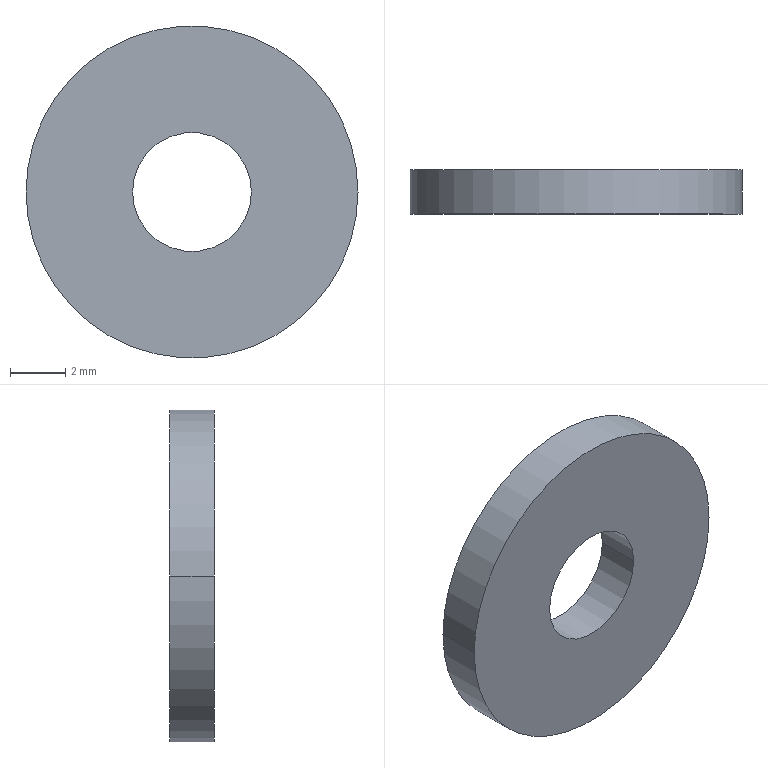Component | SolidWorks | TBN12-4-3 | 1 solid | 6 faces | box 12 x 1.6 x 12 mm | volume 158 mm3 | cylinder 4 | plane 2 | commonest cylinder face diameters 4.3 x2 12 x2
build123d program:
from build123d import *

# Parameters (mm, degrees)
SKETCH1_R           = 6
SKETCH1_R_2         = 2.15
BOSS_EXTRUDE1_DEPTH = 1.6


with BuildPart() as part:
    # Sketch1 → Boss-Extrude1 (new body)
    with BuildSketch(Plane.XY):
        Circle(SKETCH1_R)
        Circle(SKETCH1_R_2, mode=Mode.SUBTRACT)
    extrude(amount=BOSS_EXTRUDE1_DEPTH)


solid = part.part

# Placed as in the assembly
solid = solid.moved(Location((-57.536, 77.85, 217.788), (90, 0, 0)))
STEP:
#1=COLOUR_RGB('',0.7922,0.8196,0.9333);
#2=FILL_AREA_STYLE_COLOUR('',#1);
#3=FILL_AREA_STYLE('',(#2));
#4=SURFACE_STYLE_FILL_AREA(#3);
#5=SURFACE_SIDE_STYLE('',(#4));
#6=SURFACE_STYLE_USAGE(.BOTH.,#5);
#7=PRESENTATION_STYLE_ASSIGNMENT((#6));
#8=CARTESIAN_POINT('',(-2.35,3.002,8.574));
#9=VERTEX_POINT('',#8);
#10=CARTESIAN_POINT('',(-2.181,3.002,8.574));
#11=VERTEX_POINT('',#10);
#12=CARTESIAN_POINT('',(-2.265,3.002,8.574));
#13=DIRECTION('',(0.,-1.,-0.));
#14=DIRECTION('',(1.,0.,0.));
#15=AXIS2_PLACEMENT_3D('',#12,#13,#14);
#16=CIRCLE('',#15,0.08465);
#17=EDGE_CURVE('',#9,#11,#16,.T.);
#18=ORIENTED_EDGE('',*,*,#17,.T.);
#19=CARTESIAN_POINT('',(-2.181,3.065,8.574));
#20=VERTEX_POINT('',#19);
#21=CARTESIAN_POINT('',(-2.181,3.002,8.574));
#22=DIRECTION('',(-0.,1.,0.));
#23=VECTOR('',#22,39.37);
#24=LINE('',#21,#23);
#25=EDGE_CURVE('',#11,#20,#24,.T.);
#26=ORIENTED_EDGE('',*,*,#25,.T.);
#27=CARTESIAN_POINT('',(-2.35,3.065,8.574));
#28=VERTEX_POINT('',#27);
#29=CARTESIAN_POINT('',(-2.265,3.065,8.574));
#30=DIRECTION('',(0.,-1.,-0.));
#31=DIRECTION('',(1.,0.,0.));
#32=AXIS2_PLACEMENT_3D('',#29,#30,#31);
#33=CIRCLE('',#32,0.08465);
#34=EDGE_CURVE('',#28,#20,#33,.T.);
#35=ORIENTED_EDGE('',*,*,#34,.F.);
#36=CARTESIAN_POINT('',(-2.35,3.002,8.574));
#37=DIRECTION('',(-0.,1.,0.));
#38=VECTOR('',#37,39.37);
#39=LINE('',#36,#38);
#40=EDGE_CURVE('',#9,#28,#39,.T.);
#41=ORIENTED_EDGE('',*,*,#40,.F.);
#42=EDGE_LOOP('',(#18,#26,#35,#41));
#43=FACE_OUTER_BOUND('',#42,.T.);
#44=CARTESIAN_POINT('',(-2.265,3.002,8.574));
#45=DIRECTION('',(-0.,1.,0.));
#46=DIRECTION('',(-1.,0.,0.));
#47=AXIS2_PLACEMENT_3D('',#44,#45,#46);
#48=CYLINDRICAL_SURFACE('',#47,0.08465);
#49=ADVANCED_FACE('',(#43),#48,.F.);
#50=CARTESIAN_POINT('',(-2.029,3.002,8.574));
#51=VERTEX_POINT('',#50);
#52=CARTESIAN_POINT('',(-2.501,3.002,8.574));
#53=VERTEX_POINT('',#52);
#54=CARTESIAN_POINT('',(-2.265,3.002,8.574));
#55=DIRECTION('',(0.,-1.,-0.));
#56=DIRECTION('',(1.,0.,0.));
#57=AXIS2_PLACEMENT_3D('',#54,#55,#56);
#58=CIRCLE('',#57,0.2362);
#59=EDGE_CURVE('',#51,#53,#58,.T.);
#60=ORIENTED_EDGE('',*,*,#59,.F.);
#61=CARTESIAN_POINT('',(-2.029,3.065,8.574));
#62=VERTEX_POINT('',#61);
#63=CARTESIAN_POINT('',(-2.029,3.002,8.574));
#64=DIRECTION('',(-0.,1.,0.));
#65=VECTOR('',#64,39.37);
#66=LINE('',#63,#65);
#67=EDGE_CURVE('',#51,#62,#66,.T.);
#68=ORIENTED_EDGE('',*,*,#67,.T.);
#69=CARTESIAN_POINT('',(-2.501,3.065,8.574));
#70=VERTEX_POINT('',#69);
#71=CARTESIAN_POINT('',(-2.265,3.065,8.574));
#72=DIRECTION('',(0.,-1.,-0.));
#73=DIRECTION('',(1.,0.,0.));
#74=AXIS2_PLACEMENT_3D('',#71,#72,#73);
#75=CIRCLE('',#74,0.2362);
#76=EDGE_CURVE('',#62,#70,#75,.T.);
#77=ORIENTED_EDGE('',*,*,#76,.T.);
#78=CARTESIAN_POINT('',(-2.501,3.002,8.574));
#79=DIRECTION('',(-0.,1.,0.));
#80=VECTOR('',#79,39.37);
#81=LINE('',#78,#80);
#82=EDGE_CURVE('',#53,#70,#81,.T.);
#83=ORIENTED_EDGE('',*,*,#82,.F.);
#84=EDGE_LOOP('',(#60,#68,#77,#83));
#85=FACE_OUTER_BOUND('',#84,.T.);
#86=CARTESIAN_POINT('',(-2.265,3.002,8.574));
#87=DIRECTION('',(-0.,1.,0.));
#88=DIRECTION('',(-1.,0.,0.));
#89=AXIS2_PLACEMENT_3D('',#86,#87,#88);
#90=CYLINDRICAL_SURFACE('',#89,0.2362);
#91=ADVANCED_FACE('',(#85),#90,.T.);
#92=CARTESIAN_POINT('',(-2.265,3.002,8.574));
#93=DIRECTION('',(0.,-1.,-0.));
#94=DIRECTION('',(1.,0.,0.));
#95=AXIS2_PLACEMENT_3D('',#92,#93,#94);
#96=CIRCLE('',#95,0.2362);
#97=EDGE_CURVE('',#53,#51,#96,.T.);
#98=ORIENTED_EDGE('',*,*,#97,.T.);
#99=ORIENTED_EDGE('',*,*,#59,.T.);
#100=EDGE_LOOP('',(#98,#99));
#101=FACE_OUTER_BOUND('',#100,.T.);
#102=ORIENTED_EDGE('',*,*,#17,.F.);
#103=CARTESIAN_POINT('',(-2.265,3.002,8.574));
#104=DIRECTION('',(0.,-1.,-0.));
#105=DIRECTION('',(1.,0.,0.));
#106=AXIS2_PLACEMENT_3D('',#103,#104,#105);
#107=CIRCLE('',#106,0.08465);
#108=EDGE_CURVE('',#11,#9,#107,.T.);
#109=ORIENTED_EDGE('',*,*,#108,.F.);
#110=EDGE_LOOP('',(#102,#109));
#111=FACE_BOUND('',#110,.T.);
#112=CARTESIAN_POINT('',(-2.265,3.002,8.574));
#113=DIRECTION('',(0.,-1.,-0.));
#114=DIRECTION('',(1.,0.,-0.));
#115=AXIS2_PLACEMENT_3D('',#112,#113,#114);
#116=PLANE('',#115);
#117=ADVANCED_FACE('',(#101,#111),#116,.T.);
#118=CARTESIAN_POINT('',(-2.265,3.065,8.574));
#119=DIRECTION('',(0.,-1.,-0.));
#120=DIRECTION('',(1.,0.,0.));
#121=AXIS2_PLACEMENT_3D('',#118,#119,#120);
#122=CIRCLE('',#121,0.2362);
#123=EDGE_CURVE('',#70,#62,#122,.T.);
#124=ORIENTED_EDGE('',*,*,#123,.F.);
#125=ORIENTED_EDGE('',*,*,#76,.F.);
#126=EDGE_LOOP('',(#124,#125));
#127=FACE_OUTER_BOUND('',#126,.T.);
#128=ORIENTED_EDGE('',*,*,#34,.T.);
#129=CARTESIAN_POINT('',(-2.265,3.065,8.574));
#130=DIRECTION('',(0.,-1.,-0.));
#131=DIRECTION('',(1.,0.,0.));
#132=AXIS2_PLACEMENT_3D('',#129,#130,#131);
#133=CIRCLE('',#132,0.08465);
#134=EDGE_CURVE('',#20,#28,#133,.T.);
#135=ORIENTED_EDGE('',*,*,#134,.T.);
#136=EDGE_LOOP('',(#128,#135));
#137=FACE_BOUND('',#136,.T.);
#138=CARTESIAN_POINT('',(-2.265,3.065,8.574));
#139=DIRECTION('',(0.,-1.,-0.));
#140=DIRECTION('',(1.,0.,-0.));
#141=AXIS2_PLACEMENT_3D('',#138,#139,#140);
#142=PLANE('',#141);
#143=ADVANCED_FACE('',(#127,#137),#142,.F.);
#144=ORIENTED_EDGE('',*,*,#67,.F.);
#145=ORIENTED_EDGE('',*,*,#97,.F.);
#146=ORIENTED_EDGE('',*,*,#82,.T.);
#147=ORIENTED_EDGE('',*,*,#123,.T.);
#148=EDGE_LOOP('',(#144,#145,#146,#147));
#149=FACE_OUTER_BOUND('',#148,.T.);
#150=CARTESIAN_POINT('',(-2.265,3.002,8.574));
#151=DIRECTION('',(-0.,1.,0.));
#152=DIRECTION('',(-1.,0.,0.));
#153=AXIS2_PLACEMENT_3D('',#150,#151,#152);
#154=CYLINDRICAL_SURFACE('',#153,0.2362);
#155=ADVANCED_FACE('',(#149),#154,.T.);
#156=ORIENTED_EDGE('',*,*,#25,.F.);
#157=ORIENTED_EDGE('',*,*,#108,.T.);
#158=ORIENTED_EDGE('',*,*,#40,.T.);
#159=ORIENTED_EDGE('',*,*,#134,.F.);
#160=EDGE_LOOP('',(#156,#157,#158,#159));
#161=FACE_OUTER_BOUND('',#160,.T.);
#162=CARTESIAN_POINT('',(-2.265,3.002,8.574));
#163=DIRECTION('',(-0.,1.,0.));
#164=DIRECTION('',(-1.,0.,0.));
#165=AXIS2_PLACEMENT_3D('',#162,#163,#164);
#166=CYLINDRICAL_SURFACE('',#165,0.08465);
#167=ADVANCED_FACE('',(#161),#166,.F.);
#168=CLOSED_SHELL('',(#49,#91,#117,#143,#155,#167));
#169=MANIFOLD_SOLID_BREP('',#168);
#170=STYLED_ITEM('',(#7),#169);
#171=(LENGTH_UNIT()NAMED_UNIT(*)SI_UNIT($,.METRE.));
#172=LENGTH_MEASURE_WITH_UNIT(LENGTH_MEASURE(0.0254),#171);
#173=DIMENSIONAL_EXPONENTS(1.,0.,0.,0.,0.,0.,0.);
#174=(CONVERSION_BASED_UNIT('',#172)LENGTH_UNIT()NAMED_UNIT(#173));
#175=UNCERTAINTY_MEASURE_WITH_UNIT(LENGTH_MEASURE(0.00001),#174,'','');
#176=(NAMED_UNIT(*)PLANE_ANGLE_UNIT()SI_UNIT($,.RADIAN.));
#177=(NAMED_UNIT(*)SI_UNIT($,.STERADIAN.)SOLID_ANGLE_UNIT());
#178=(GEOMETRIC_REPRESENTATION_CONTEXT(3)GLOBAL_UNCERTAINTY_ASSIGNED_CONTEXT((#175))GLOBAL_UNIT_ASSIGNED_CONTEXT((#174,#176,#177))REPRESENTATION_CONTEXT('',''));
#179=MECHANICAL_DESIGN_GEOMETRIC_PRESENTATION_REPRESENTATION('',(#170),#178);
#180=CARTESIAN_POINT('',(0.,0.,0.));
#181=DIRECTION('',(0.,0.,1.));
#182=DIRECTION('',(1.,0.,0.));
#183=AXIS2_PLACEMENT_3D('',#180,#181,#182);
#184=(LENGTH_UNIT()NAMED_UNIT(*)SI_UNIT($,.METRE.));
#185=LENGTH_MEASURE_WITH_UNIT(LENGTH_MEASURE(0.0254),#184);
#186=DIMENSIONAL_EXPONENTS(1.,0.,0.,0.,0.,0.,0.);
#187=(CONVERSION_BASED_UNIT('',#185)LENGTH_UNIT()NAMED_UNIT(#186));
#188=UNCERTAINTY_MEASURE_WITH_UNIT(LENGTH_MEASURE(0.00001),#187,'','');
#189=(NAMED_UNIT(*)PLANE_ANGLE_UNIT()SI_UNIT($,.RADIAN.));
#190=(NAMED_UNIT(*)SI_UNIT($,.STERADIAN.)SOLID_ANGLE_UNIT());
#191=(GEOMETRIC_REPRESENTATION_CONTEXT(3)GLOBAL_UNCERTAINTY_ASSIGNED_CONTEXT((#188))GLOBAL_UNIT_ASSIGNED_CONTEXT((#187,#189,#190))REPRESENTATION_CONTEXT('',''));
#192=ADVANCED_BREP_SHAPE_REPRESENTATION('',(#169,#183),#191);
#193=PRESENTATION_LAYER_ASSIGNMENT('','',(#170));